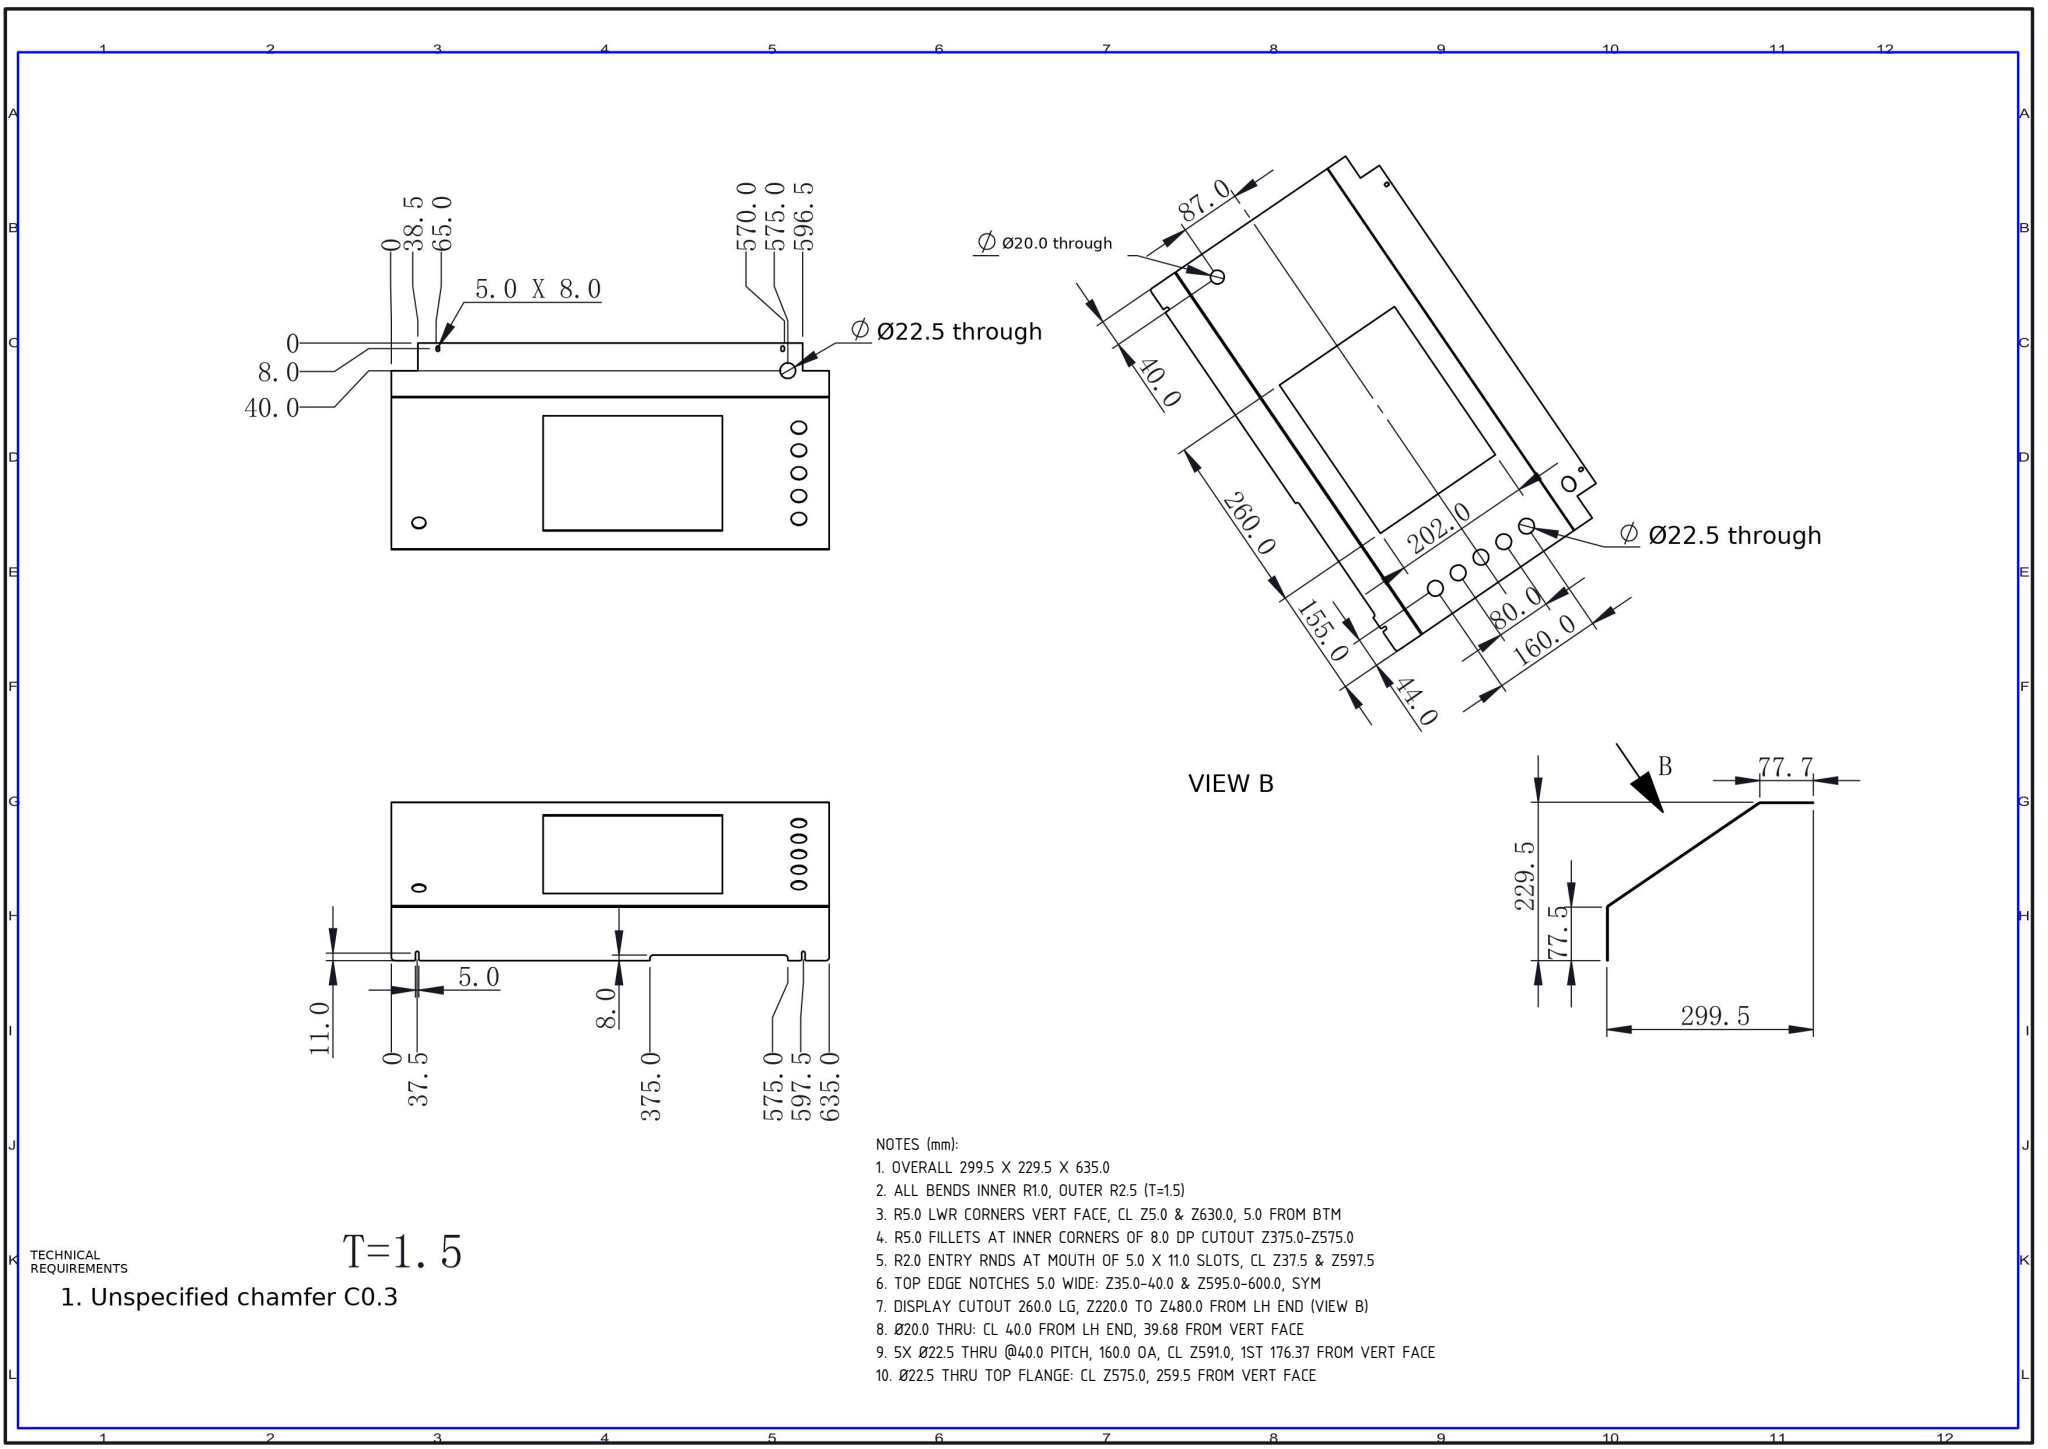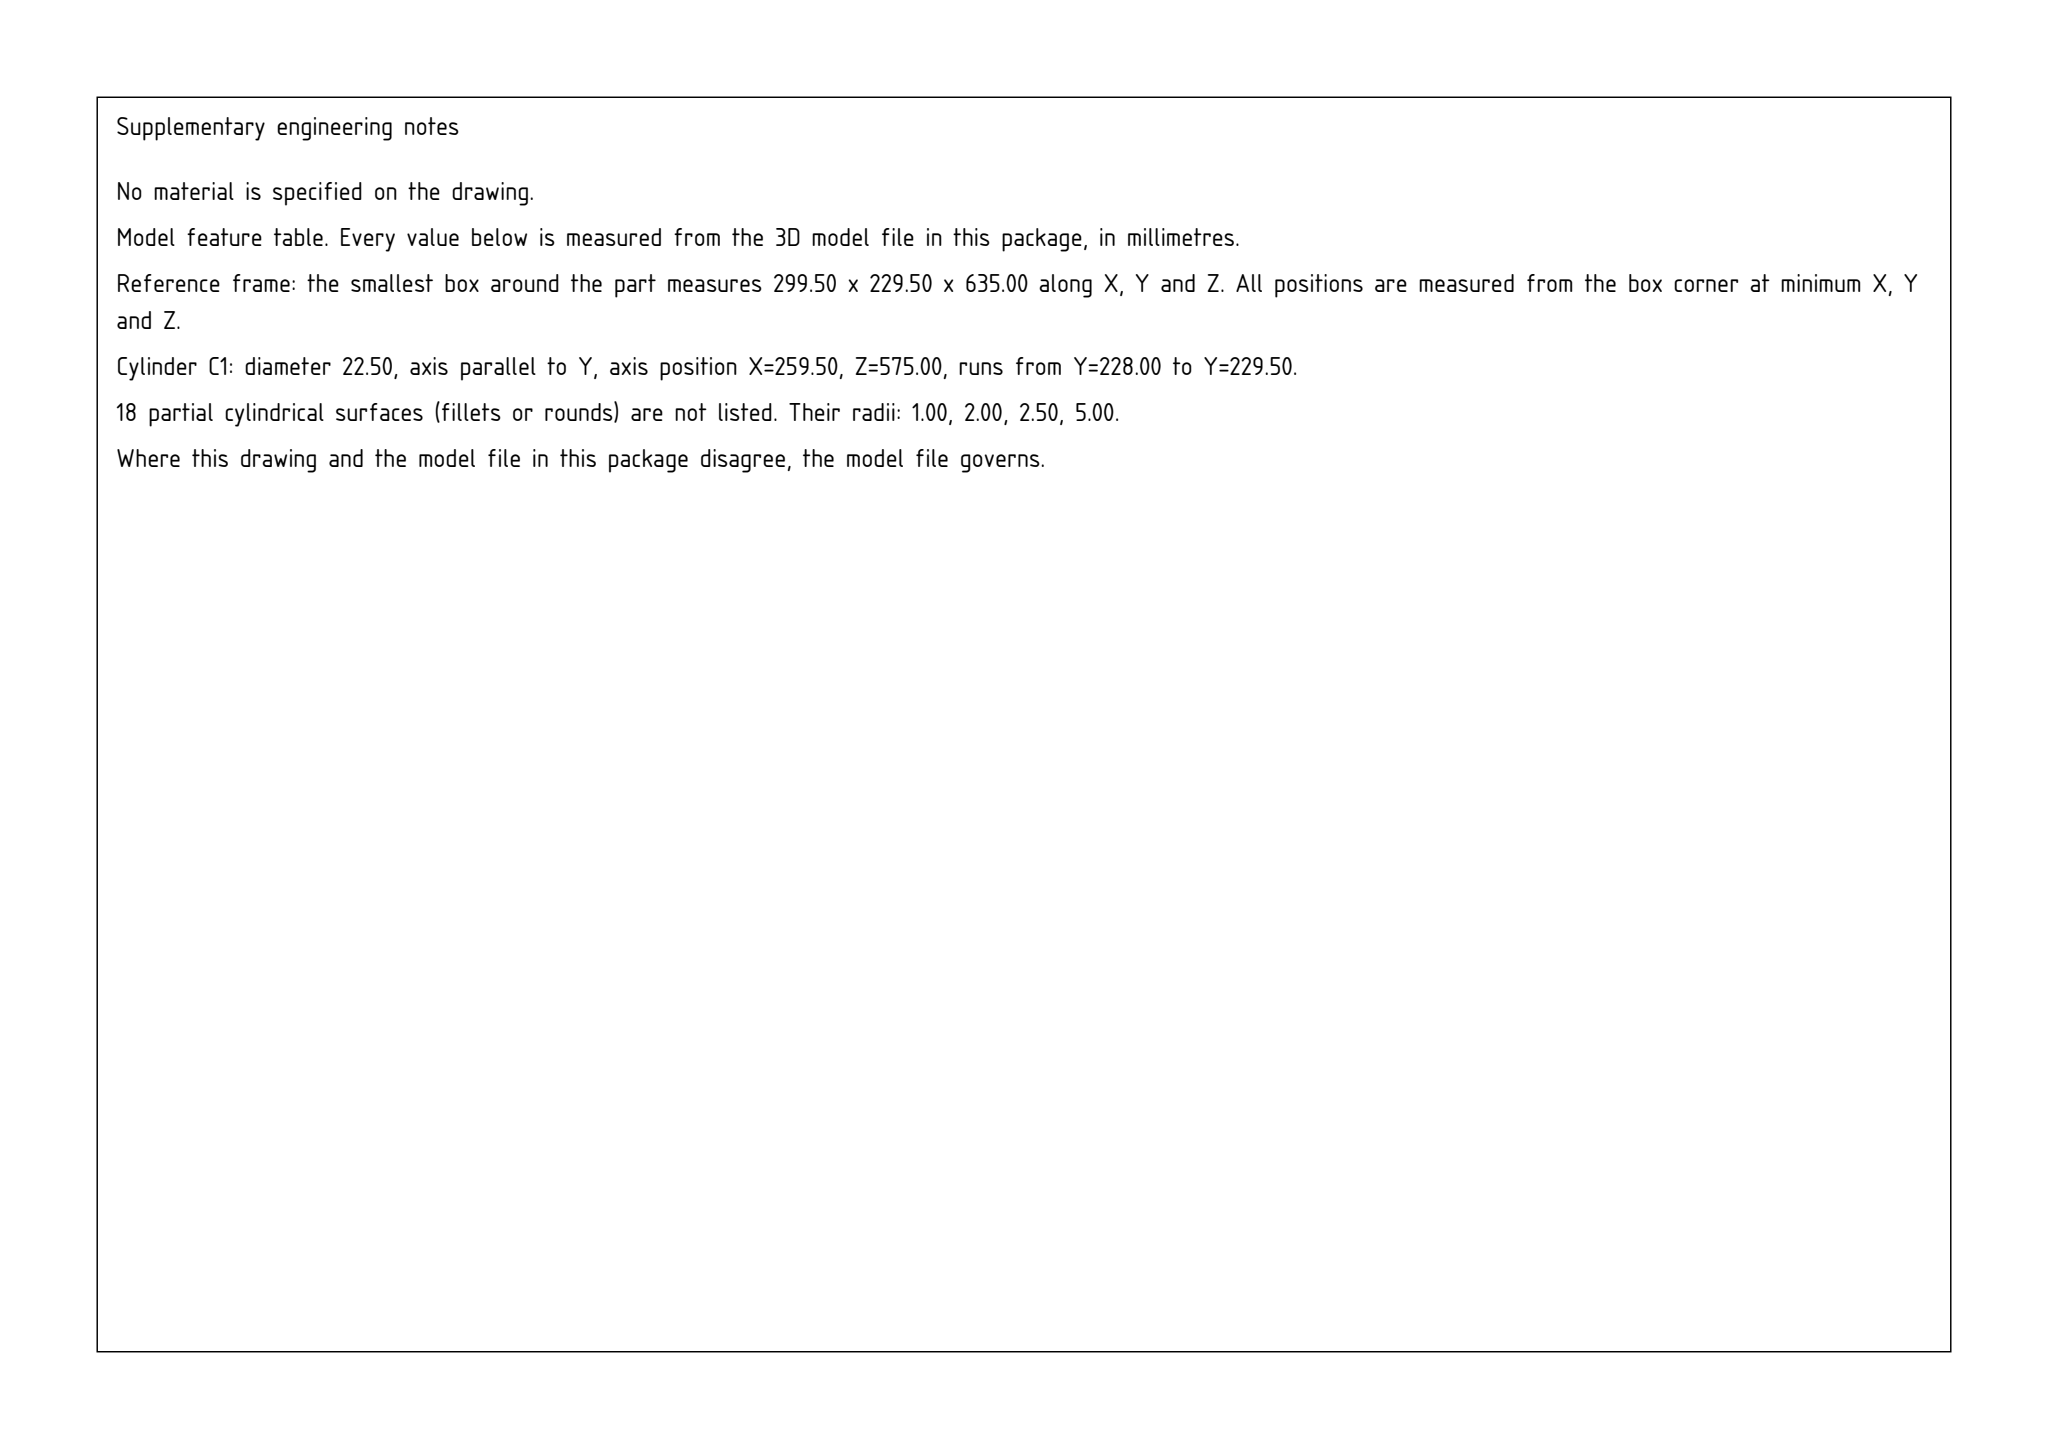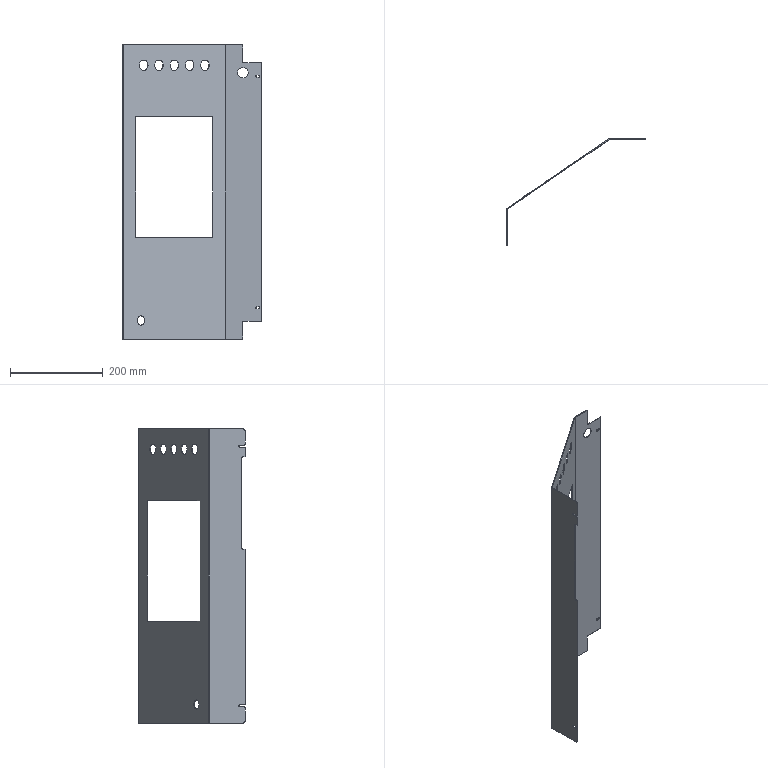Part | SolidWorks | mm | 1 solid | 72 faces | box 299.5 x 229.5 x 635 mm | volume 313083 mm3 | plane 40 | cylinder 32 | commonest cylinder face diameters 22.5 x12 5 x8 10 x4 4 x4 20 x2 2 x2
Drawing notes:
OVERALL 299.5 X 229.5 X 635.0 | from the solid: bbox_xyz [299.5, 229.5, 635.0]
ALL BENDS INNER R1.0, OUTER R2.5 (T=1.5) | from the solid: z-axis cyls dia 2.0 & 5.0 at (2.5,77.47) and (221.81,227.0), L=635.0
R5.0 LWR CORNERS VERT FACE, CL Z5.0 & Z630.0, 5.0 FROM BTM | from the solid: x-axis cyls dia 10.0 at (y5.0,z5.0) and (y5.0,z630.0), L=1.5
R5.0 FILLETS AT INNER CORNERS OF 8.0 DP CUTOUT Z375.0-Z575.0 | from the solid: x-axis cyls dia 10.0 at (y3.0,z380.0) and (y3.0,z570.0), L=1.5
R2.0 ENTRY RNDS AT MOUTH OF 5.0 X 11.0 SLOTS, CL Z37.5 & Z597.5 | from the solid: x-axis cyls dia 4.0 at y2.0, z33.0/42.0 & z593.0/602.0, L=1.5
TOP EDGE NOTCHES 5.0 WIDE: Z35.0-40.0 & Z595.0-600.0, SYM | from the solid: z-planes 35.0/40.0 and 595.0/600.0, mirrored about 317.5 of 635.0 lg
DISPLAY CUTOUT 260.0 LG, Z220.0 TO Z480.0 FROM LH END (VIEW B) | from the solid: z-planes 220.0 and 480.0 bound cutout: 480.0-220.0 = 260.0 lg
Ø20.0 THRU: CL 40.0 FROM LH END, 39.68 FROM VERT FACE | from the solid: cylinder [20.0,'y',[39.68,null,40.0],12.51] thru sloped face
5X Ø22.5 THRU @40.0 PITCH, 160.0 OA, CL Z591.0, 1ST 176.37 FROM VERT FACE | from the solid: 22.5 dia y-cyls at z=591.0, x=176.37/209.42/242.47/275.52/308.56; dX 33.05 = 40.0 on slope
Ø22.5 THRU TOP FLANGE: CL Z575.0, 259.5 FROM VERT FACE | from the solid: cylinder [22.5,'y',[259.5,null,575.0],1.5] in 1.5 thk y-normal flange